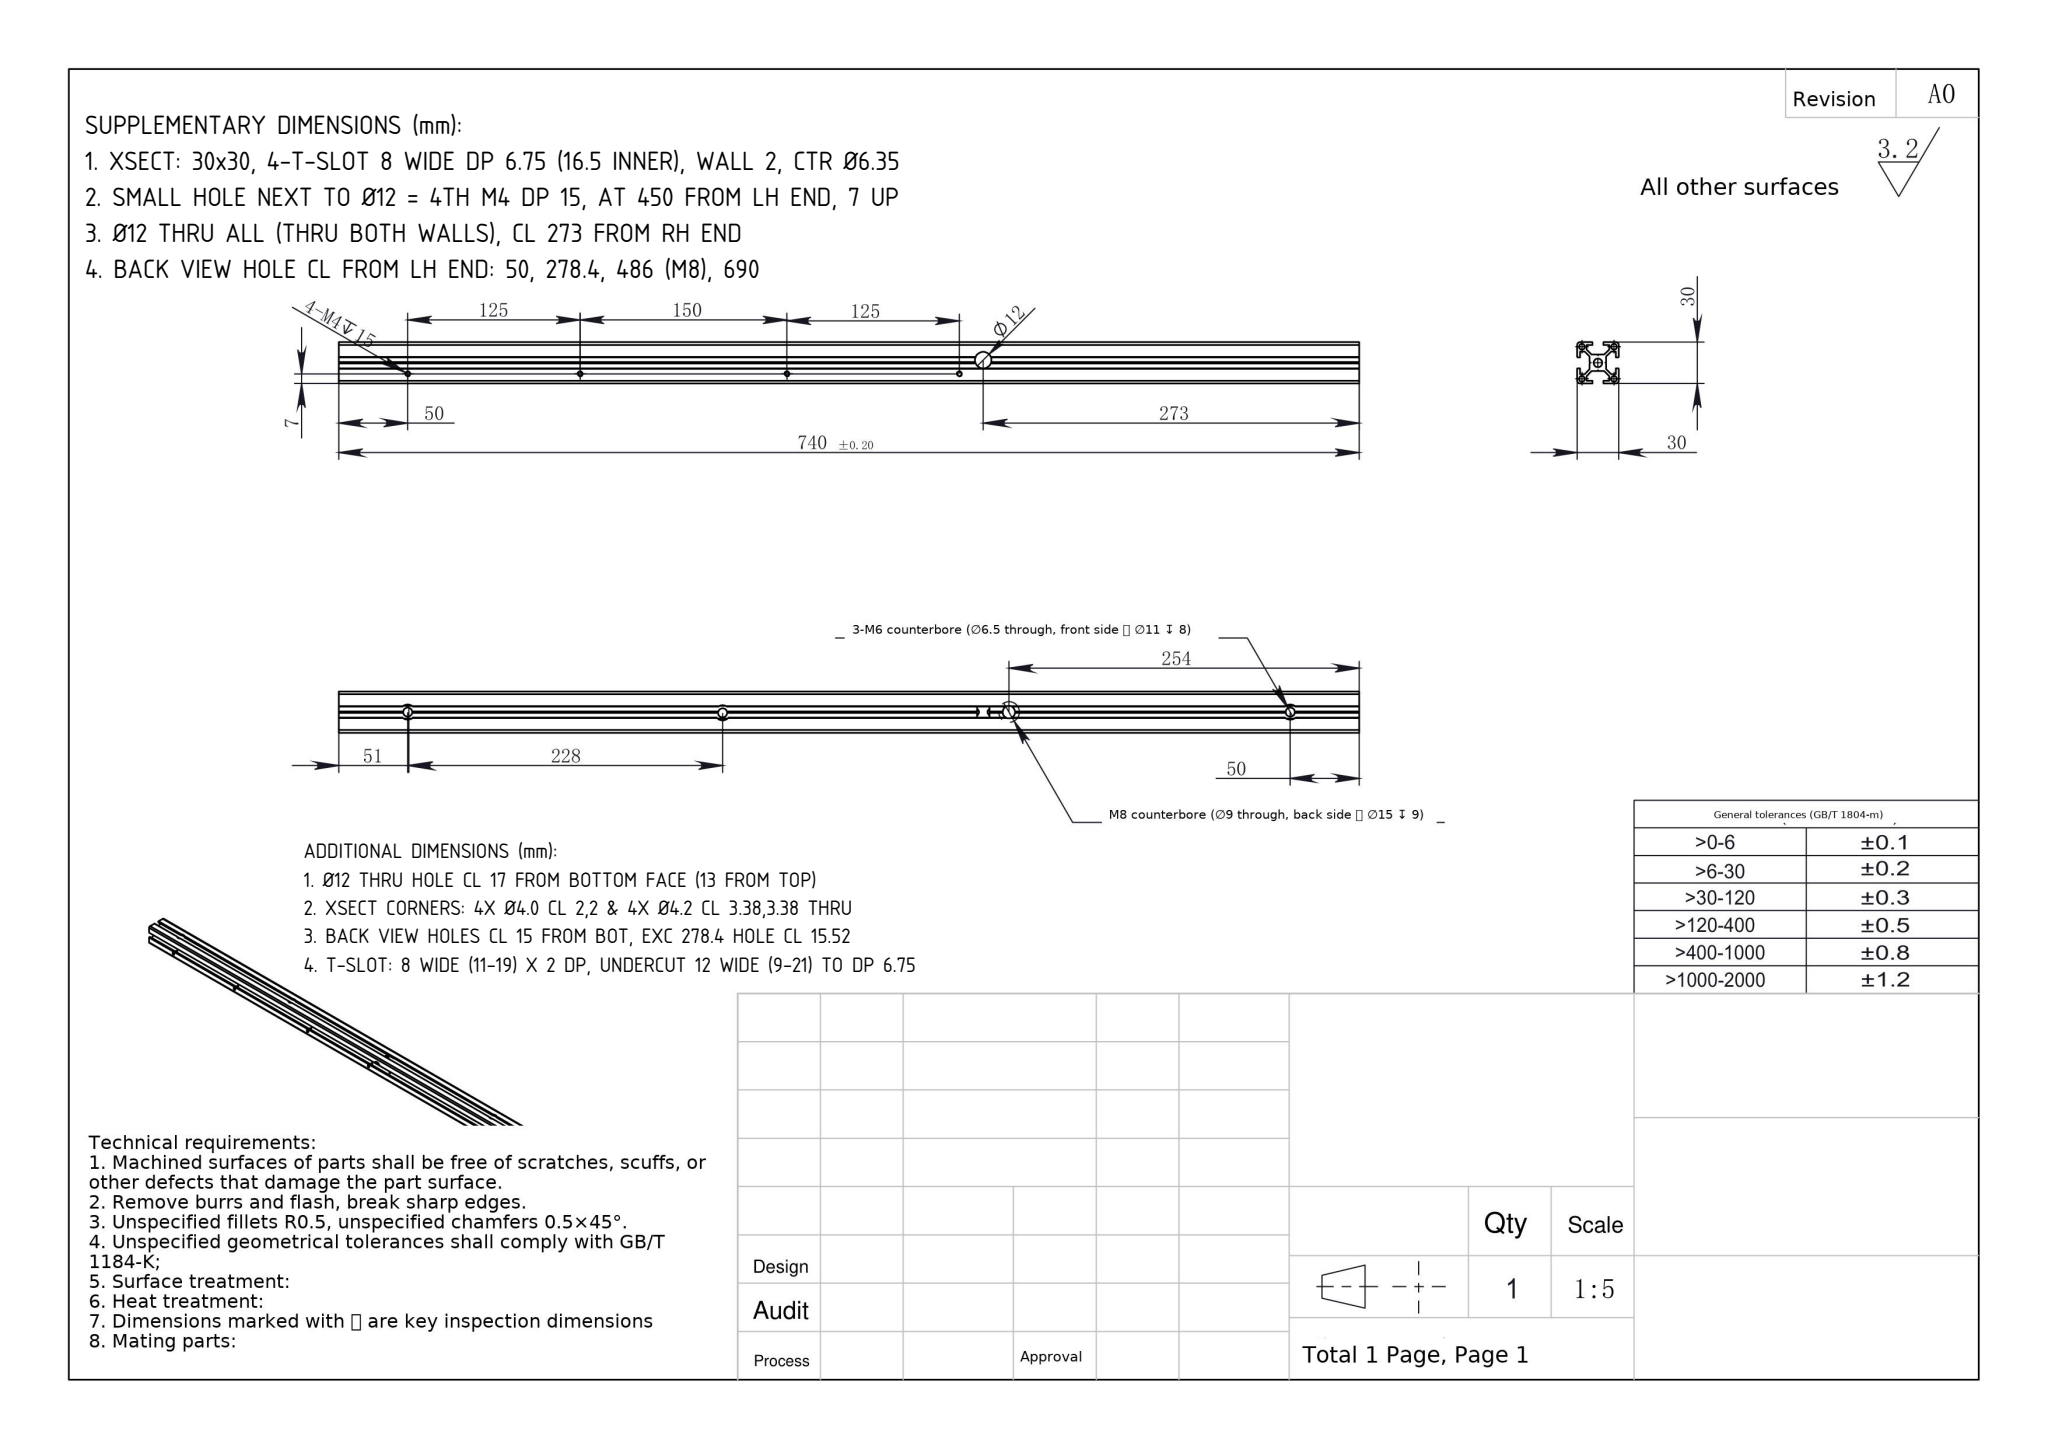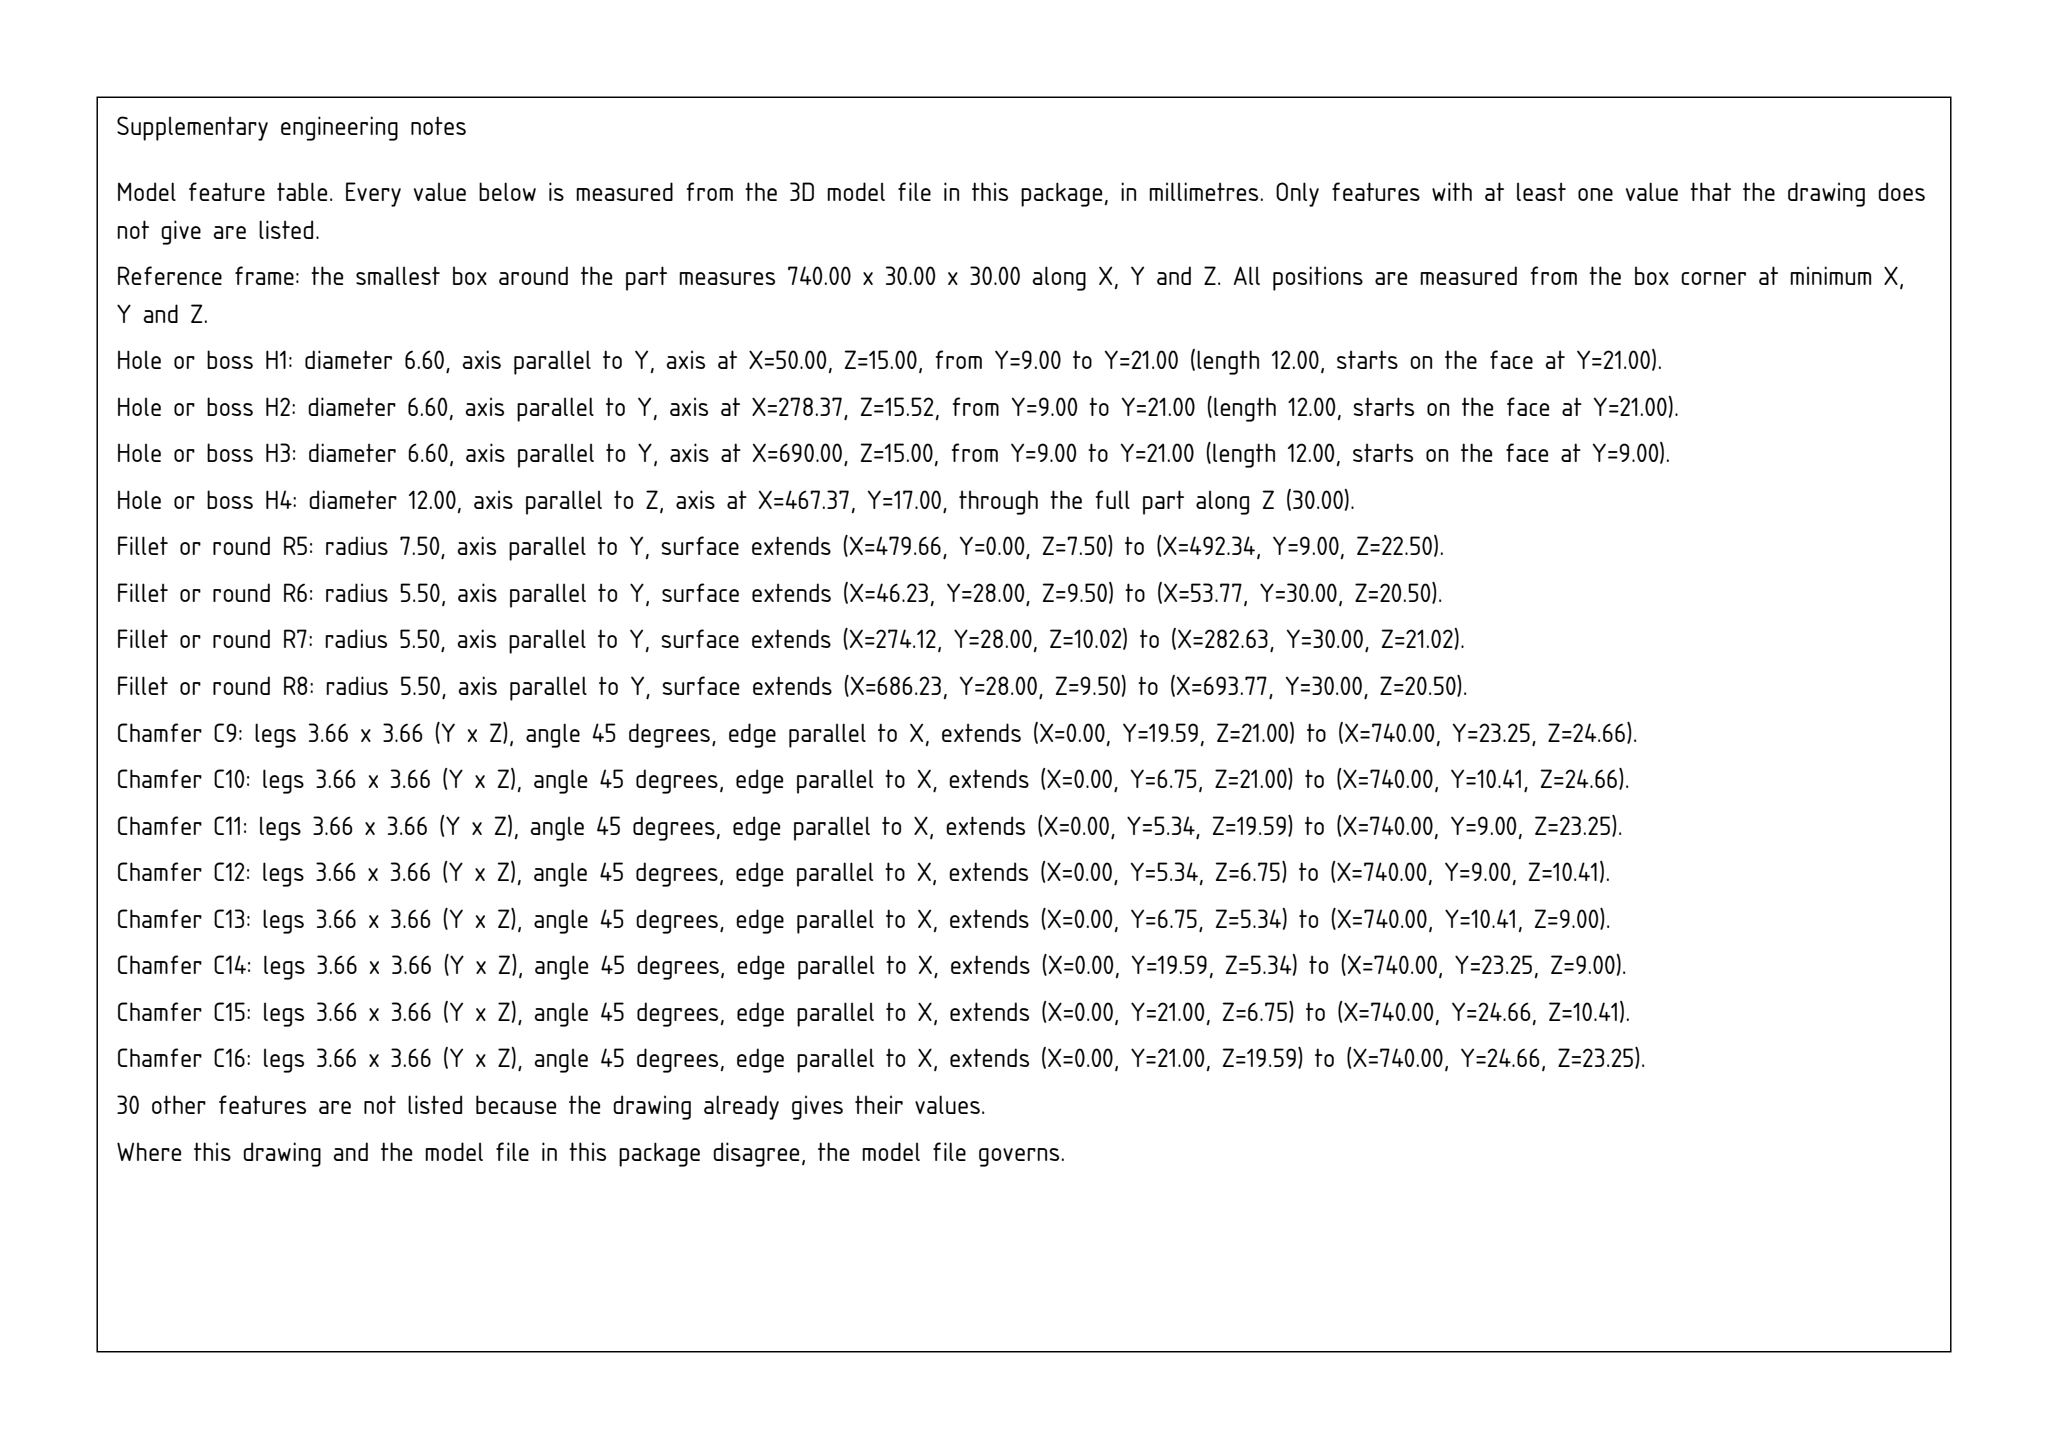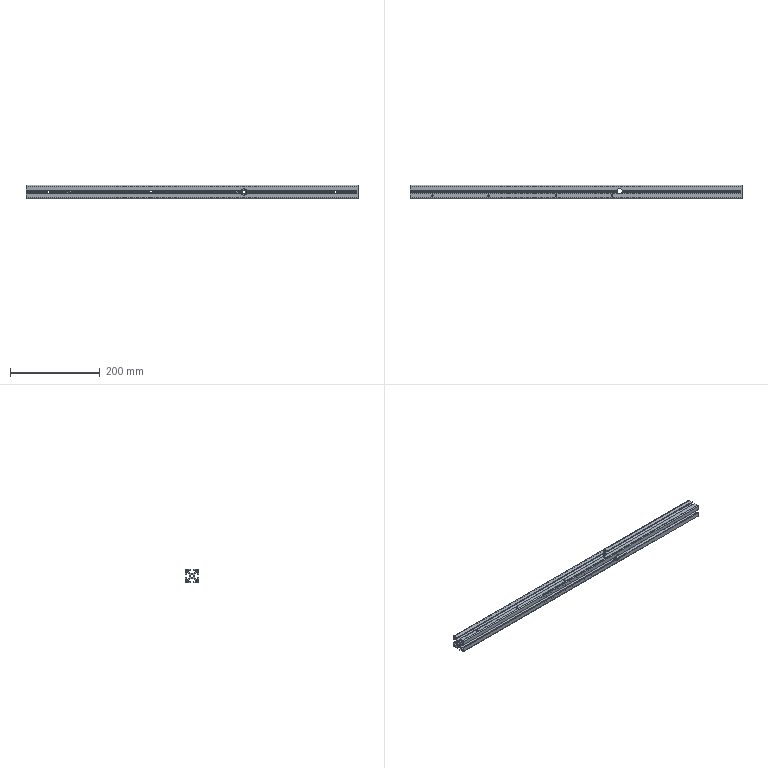Part | SolidWorks | mm | 1 solid | 184 faces | box 740 x 30 x 30 mm | volume 246220 mm3 | plane 100 | cylinder 84 | commonest cylinder face diameters 0.6 x20 3.3 x12 6.346 x10 11 x9 4.2 x8 15 x6 6.6 x6 9 x5
build123d program:
from build123d import *

# Parameters (mm, degrees)
SKETCH1_2_R                                          = 2.1
SKETCH1_2_R_2                                        = 3.173
BOSS_EXTRUDE1_DEPTH                                  = 740
SKETCH1_R                                            = 6
CUT_EXTRUDE1_DEPTH                                   = 742.656
M4_TAPPED_HOLE1_D                                    = 3.3
M4_TAPPED_HOLE1_DEPTH                                = 18.5
M4_TAPPED_HOLE1_TIP                                  = 0.9914
CBORE_FOR_M6_HEXAGON_SOCKET_HEAD_CAP_SCR_D           = 6.6
CBORE_FOR_M6_HEXAGON_SOCKET_HEAD_CAP_SCR_DEPTH       = 45
CBORE_FOR_M6_HEXAGON_SOCKET_HEAD_CAP_SCR_CBORE_D     = 11
CBORE_FOR_M6_HEXAGON_SOCKET_HEAD_CAP_SCR_CBORE_DEPTH = 6.8
CBORE_FOR_M6_HEXAGON_SOCKET_HEAD_CAP_SCR_TIP         = 1.983
CBORE_FOR_M8_HEXAGON_SOCKET_HEAD_CAP_SCR_D           = 9
CBORE_FOR_M8_HEXAGON_SOCKET_HEAD_CAP_SCR_DEPTH       = 40
CBORE_FOR_M8_HEXAGON_SOCKET_HEAD_CAP_SCR_CBORE_D     = 15
CBORE_FOR_M8_HEXAGON_SOCKET_HEAD_CAP_SCR_CBORE_DEPTH = 9
CBORE_FOR_M8_HEXAGON_SOCKET_HEAD_CAP_SCR_TIP         = 2.704


with BuildPart() as part:
    # Sketch1_2 → Boss-Extrude1 (new body)
    with BuildSketch(Plane(origin=(0, 0, 0), x_dir=(0, 0, -1), z_dir=(1, 0, 0))):
        with BuildLine():
            Line((5.112, 37.423), (5.112, 28.723))
            ThreePointArc((5.112, 28.723), (5.2, 28.511), (5.412, 28.423))
            Line((5.412, 28.423), (7.112, 28.423))
            Line((7.112, 28.423), (7.112, 32.673))
            Line((7.112, 32.673), (10.448, 32.673))
            Line((10.448, 32.673), (14.112, 29.009))
            Line((14.112, 29.009), (14.112, 24.943))
            Line((14.112, 24.943), (14.412, 24.423))
            Line((14.412, 24.423), (14.112, 23.904))
            Line((14.112, 23.904), (14.112, 19.837))
            Line((14.112, 19.837), (10.448, 16.173))
            Line((10.448, 16.173), (7.112, 16.173))
            Line((7.112, 16.173), (7.112, 20.423))
            Line((7.112, 20.423), (5.412, 20.423))
            ThreePointArc((5.412, 20.423), (5.2, 20.335), (5.112, 20.123))
            Line((5.112, 20.123), (5.112, 11.423))
            ThreePointArc((5.112, 11.423), (5.698, 10.009), (7.112, 9.423))
            Line((7.112, 9.423), (15.812, 9.423))
            ThreePointArc((15.812, 9.423), (16.024, 9.511), (16.112, 9.723))
            Line((16.112, 9.723), (16.112, 11.423))
            Line((16.112, 11.423), (11.862, 11.423))
            Line((11.862, 11.423), (11.862, 14.759))
            Line((11.862, 14.759), (15.526, 18.423))
            Line((15.526, 18.423), (19.592, 18.423))
            Line((19.592, 18.423), (20.112, 18.723))
            Line((20.112, 18.723), (20.631, 18.423))
            Line((20.631, 18.423), (24.698, 18.423))
            Line((24.698, 18.423), (28.362, 14.759))
            Line((28.362, 14.759), (28.362, 11.423))
            Line((28.362, 11.423), (24.112, 11.423))
            Line((24.112, 11.423), (24.112, 9.723))
            ThreePointArc((24.112, 9.723), (24.2, 9.511), (24.412, 9.423))
            Line((24.412, 9.423), (33.112, 9.423))
            ThreePointArc((33.112, 9.423), (34.526, 10.009), (35.112, 11.423))
            Line((35.112, 11.423), (35.112, 20.123))
            ThreePointArc((35.112, 20.123), (35.024, 20.335), (34.812, 20.423))
            Line((34.812, 20.423), (33.112, 20.423))
            Line((33.112, 20.423), (33.112, 16.173))
            Line((33.112, 16.173), (29.776, 16.173))
            Line((29.776, 16.173), (26.112, 19.837))
            Line((26.112, 19.837), (26.112, 23.904))
            Line((26.112, 23.904), (25.812, 24.423))
            Line((25.812, 24.423), (26.112, 24.943))
            Line((26.112, 24.943), (26.112, 29.009))
            Line((26.112, 29.009), (29.776, 32.673))
            Line((29.776, 32.673), (33.112, 32.673))
            Line((33.112, 32.673), (33.112, 28.423))
            Line((33.112, 28.423), (34.812, 28.423))
            ThreePointArc((34.812, 28.423), (35.024, 28.511), (35.112, 28.723))
            Line((35.112, 28.723), (35.112, 37.423))
            ThreePointArc((35.112, 37.423), (34.526, 38.837), (33.112, 39.423))
            Line((33.112, 39.423), (24.412, 39.423))
            ThreePointArc((24.412, 39.423), (24.2, 39.335), (24.112, 39.123))
            Line((24.112, 39.123), (24.112, 37.423))
            Line((24.112, 37.423), (28.362, 37.423))
            Line((28.362, 37.423), (28.362, 34.087))
            Line((28.362, 34.087), (24.698, 30.423))
            Line((24.698, 30.423), (20.631, 30.423))
            Line((20.631, 30.423), (20.112, 30.123))
            Line((20.112, 30.123), (19.592, 30.423))
            Line((19.592, 30.423), (15.526, 30.423))
            Line((15.526, 30.423), (11.862, 34.087))
            Line((11.862, 34.087), (11.862, 37.423))
            Line((11.862, 37.423), (16.112, 37.423))
            Line((16.112, 37.423), (16.112, 39.123))
            ThreePointArc((16.112, 39.123), (16.024, 39.335), (15.812, 39.423))
            Line((15.812, 39.423), (7.112, 39.423))
            ThreePointArc((7.112, 39.423), (5.698, 38.837), (5.112, 37.423))
        make_face()
        with Locations((31.737, 12.798)):
            Circle(SKETCH1_2_R, mode=Mode.SUBTRACT)
        with Locations((31.737, 36.048)):
            Circle(SKETCH1_2_R, mode=Mode.SUBTRACT)
        with Locations((8.487, 12.798)):
            Circle(SKETCH1_2_R, mode=Mode.SUBTRACT)
        with Locations((8.487, 36.048)):
            Circle(SKETCH1_2_R, mode=Mode.SUBTRACT)
        with Locations((20.112, 24.423)):
            Circle(SKETCH1_2_R_2, mode=Mode.SUBTRACT)
    extrude(amount=BOSS_EXTRUDE1_DEPTH)

    # Sketch1 → Cut-Extrude1 (cut, through all)
    with BuildSketch(Plane.XY.offset(-5.112)):
        with Locations(Location((467.374, 26.423, 0), (0, 0, 345.716))):
            Circle(SKETCH1_R)
    extrude(amount=-CUT_EXTRUDE1_DEPTH, mode=Mode.SUBTRACT)

    # M4 Tapped Hole1
    with Locations(Plane.XY.offset(-5.112)):
        with Locations((50, 16.423), (175, 16.423), (325, 16.423), (450, 16.423)):
            Hole(M4_TAPPED_HOLE1_D / 2, depth=M4_TAPPED_HOLE1_DEPTH)
            with Locations((0, 0, -(M4_TAPPED_HOLE1_DEPTH + M4_TAPPED_HOLE1_TIP / 2))):  # 118° drill point
                Cone(0, M4_TAPPED_HOLE1_D / 2, M4_TAPPED_HOLE1_TIP, mode=Mode.SUBTRACT)

    # CBORE for M6 Hexagon socket head cap scr
    with Locations(Plane(origin=(0, 39.423, 0), x_dir=(1, 0, 0), z_dir=(0, 1, 0))):
        with Locations((690, 20.112), (278.374, 19.592), (50, 20.112)):
            CounterBoreHole(CBORE_FOR_M6_HEXAGON_SOCKET_HEAD_CAP_SCR_D / 2, CBORE_FOR_M6_HEXAGON_SOCKET_HEAD_CAP_SCR_CBORE_D / 2, CBORE_FOR_M6_HEXAGON_SOCKET_HEAD_CAP_SCR_CBORE_DEPTH, depth=CBORE_FOR_M6_HEXAGON_SOCKET_HEAD_CAP_SCR_DEPTH)
            with Locations((0, 0, -(CBORE_FOR_M6_HEXAGON_SOCKET_HEAD_CAP_SCR_DEPTH + CBORE_FOR_M6_HEXAGON_SOCKET_HEAD_CAP_SCR_TIP / 2))):  # 118° drill point
                Cone(0, CBORE_FOR_M6_HEXAGON_SOCKET_HEAD_CAP_SCR_D / 2, CBORE_FOR_M6_HEXAGON_SOCKET_HEAD_CAP_SCR_TIP, mode=Mode.SUBTRACT)

    # CBORE for M8 Hexagon socket head cap scr
    with Locations(Plane(origin=(0, 9.423, 0), x_dir=(-1, 0, 0), z_dir=(0, -1, 0))):
        with Locations((-486, 20.112)):
            CounterBoreHole(CBORE_FOR_M8_HEXAGON_SOCKET_HEAD_CAP_SCR_D / 2, CBORE_FOR_M8_HEXAGON_SOCKET_HEAD_CAP_SCR_CBORE_D / 2, CBORE_FOR_M8_HEXAGON_SOCKET_HEAD_CAP_SCR_CBORE_DEPTH, depth=CBORE_FOR_M8_HEXAGON_SOCKET_HEAD_CAP_SCR_DEPTH)
            with Locations((0, 0, -(CBORE_FOR_M8_HEXAGON_SOCKET_HEAD_CAP_SCR_DEPTH + CBORE_FOR_M8_HEXAGON_SOCKET_HEAD_CAP_SCR_TIP / 2))):  # 118° drill point
                Cone(0, CBORE_FOR_M8_HEXAGON_SOCKET_HEAD_CAP_SCR_D / 2, CBORE_FOR_M8_HEXAGON_SOCKET_HEAD_CAP_SCR_TIP, mode=Mode.SUBTRACT)


solid = part.part